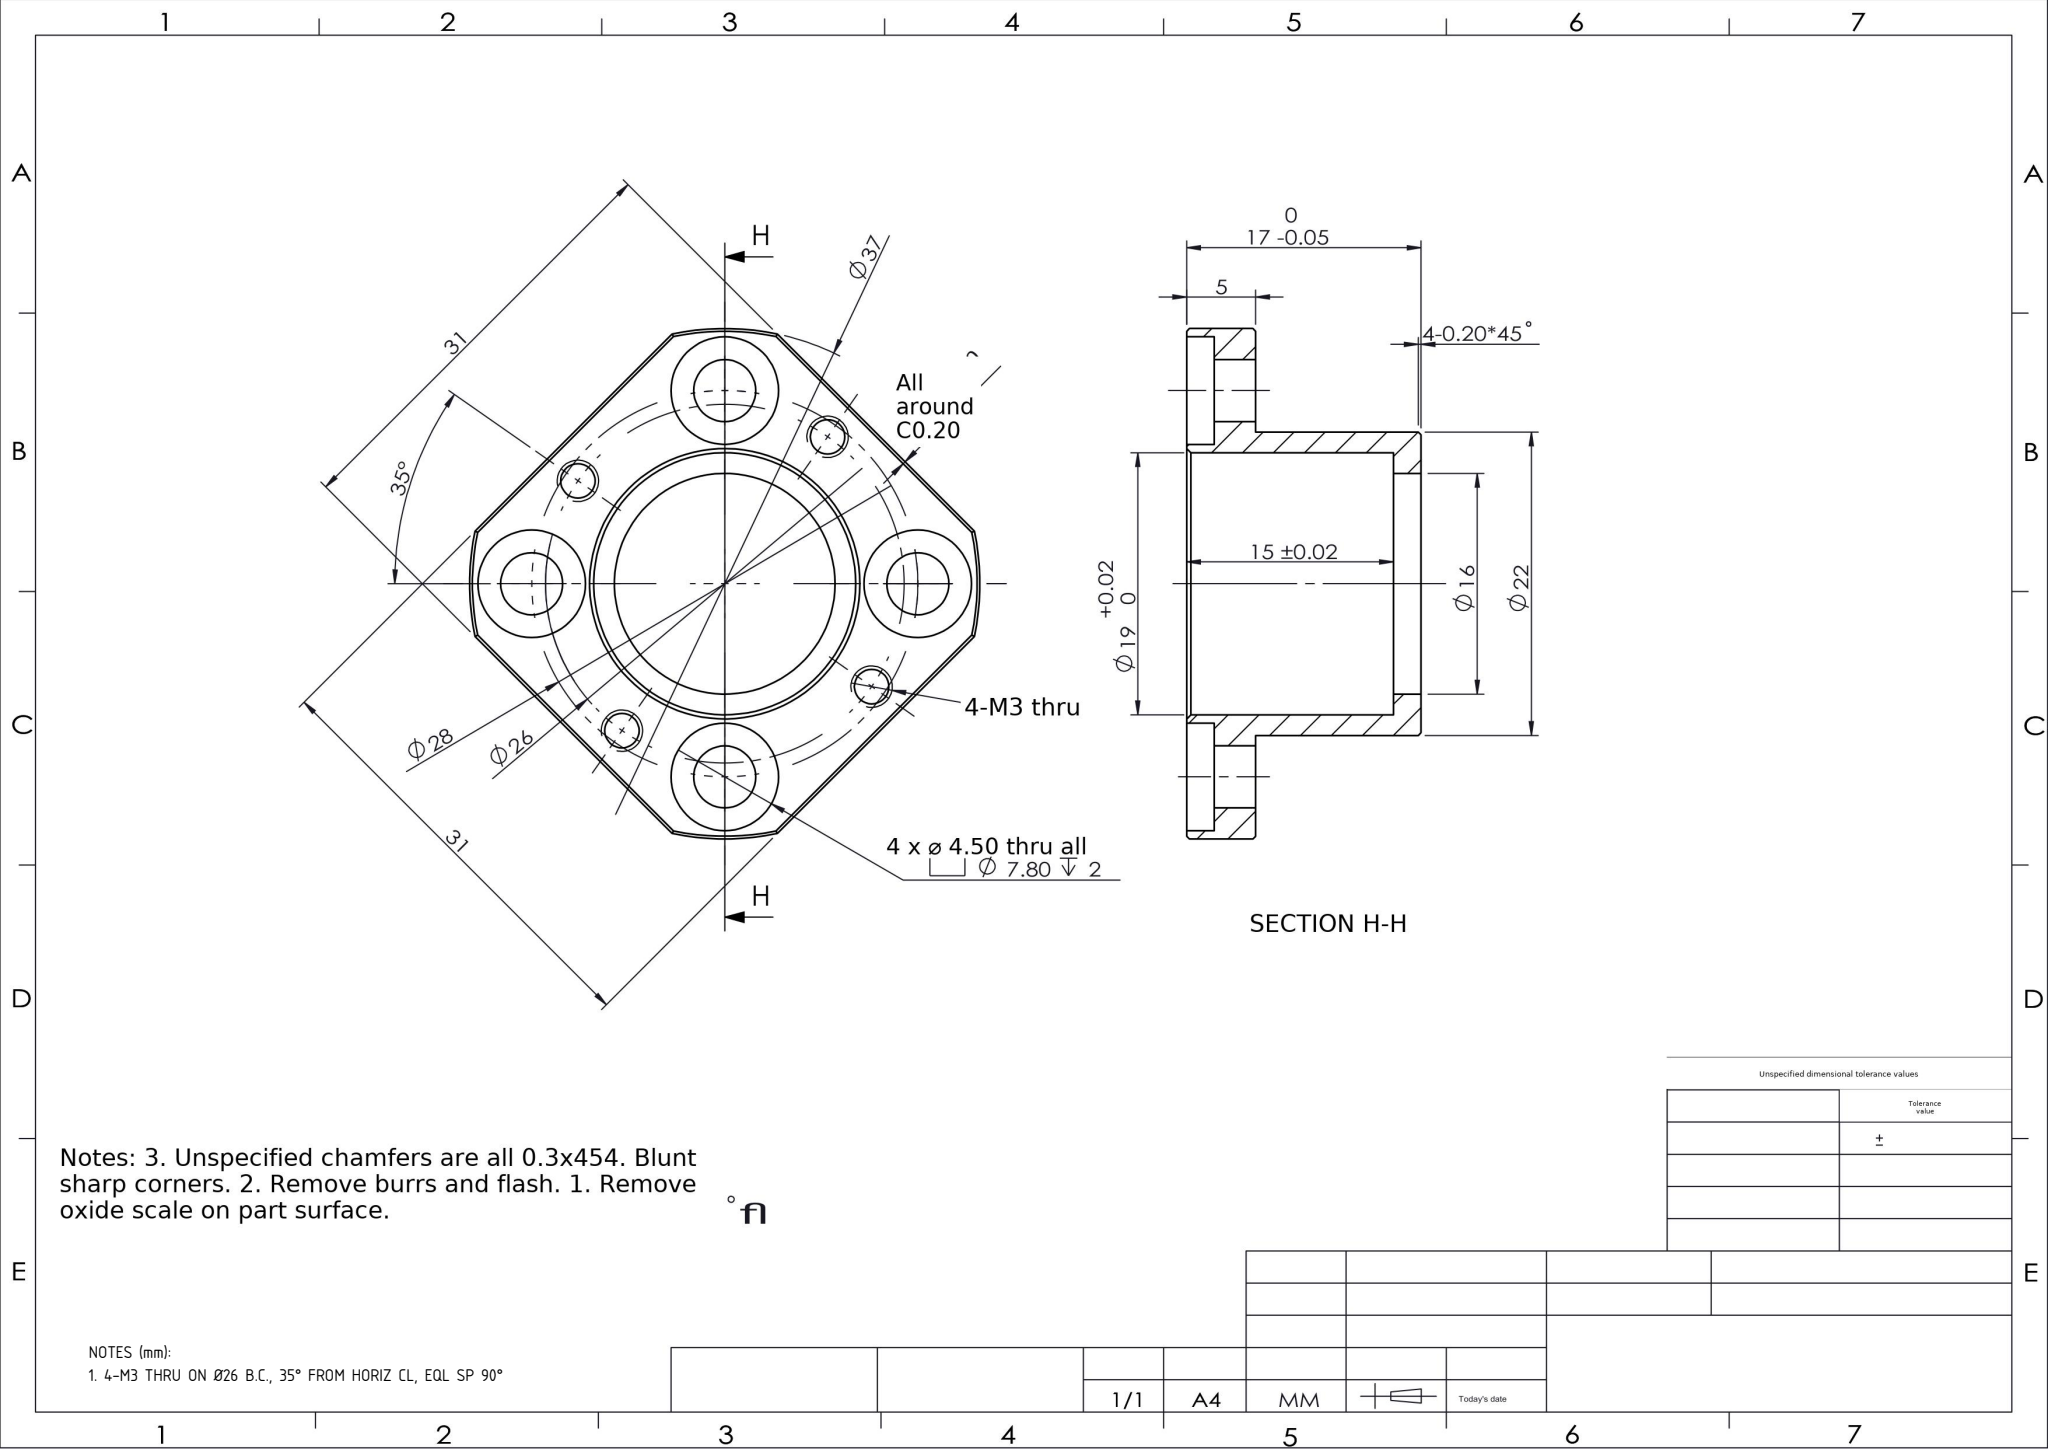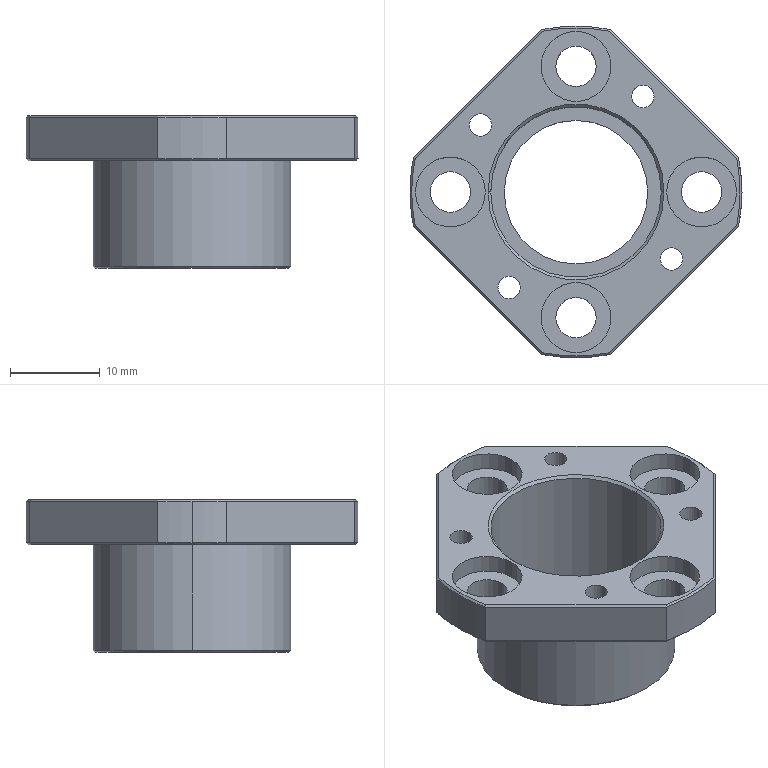Part | SolidWorks | mm | 1 solid | 69 faces | box 37 x 37 x 17 mm | volume 3781 mm3 | cylinder 35 | plane 20 | cone 14 | commonest cylinder face diameters 2.5 x8 7.8 x8 4.5 x8 37 x5 19 x2 22 x2 16 x2
Drawing notes:
4-M3 THRU ON Ø26 B.C., 35° FROM HORIZ CL, EQL SP 90° | from the solid: Ø2.5 holes at (7.85,25.96),(11.04,7.85),(25.96,29.15),(29.15,11.04) about center (18.5,18.5): R=13.0 (Ø26 B.C.), angles 55°/145°/235°/325°, i.e. 35° from X centerline, 90° apart